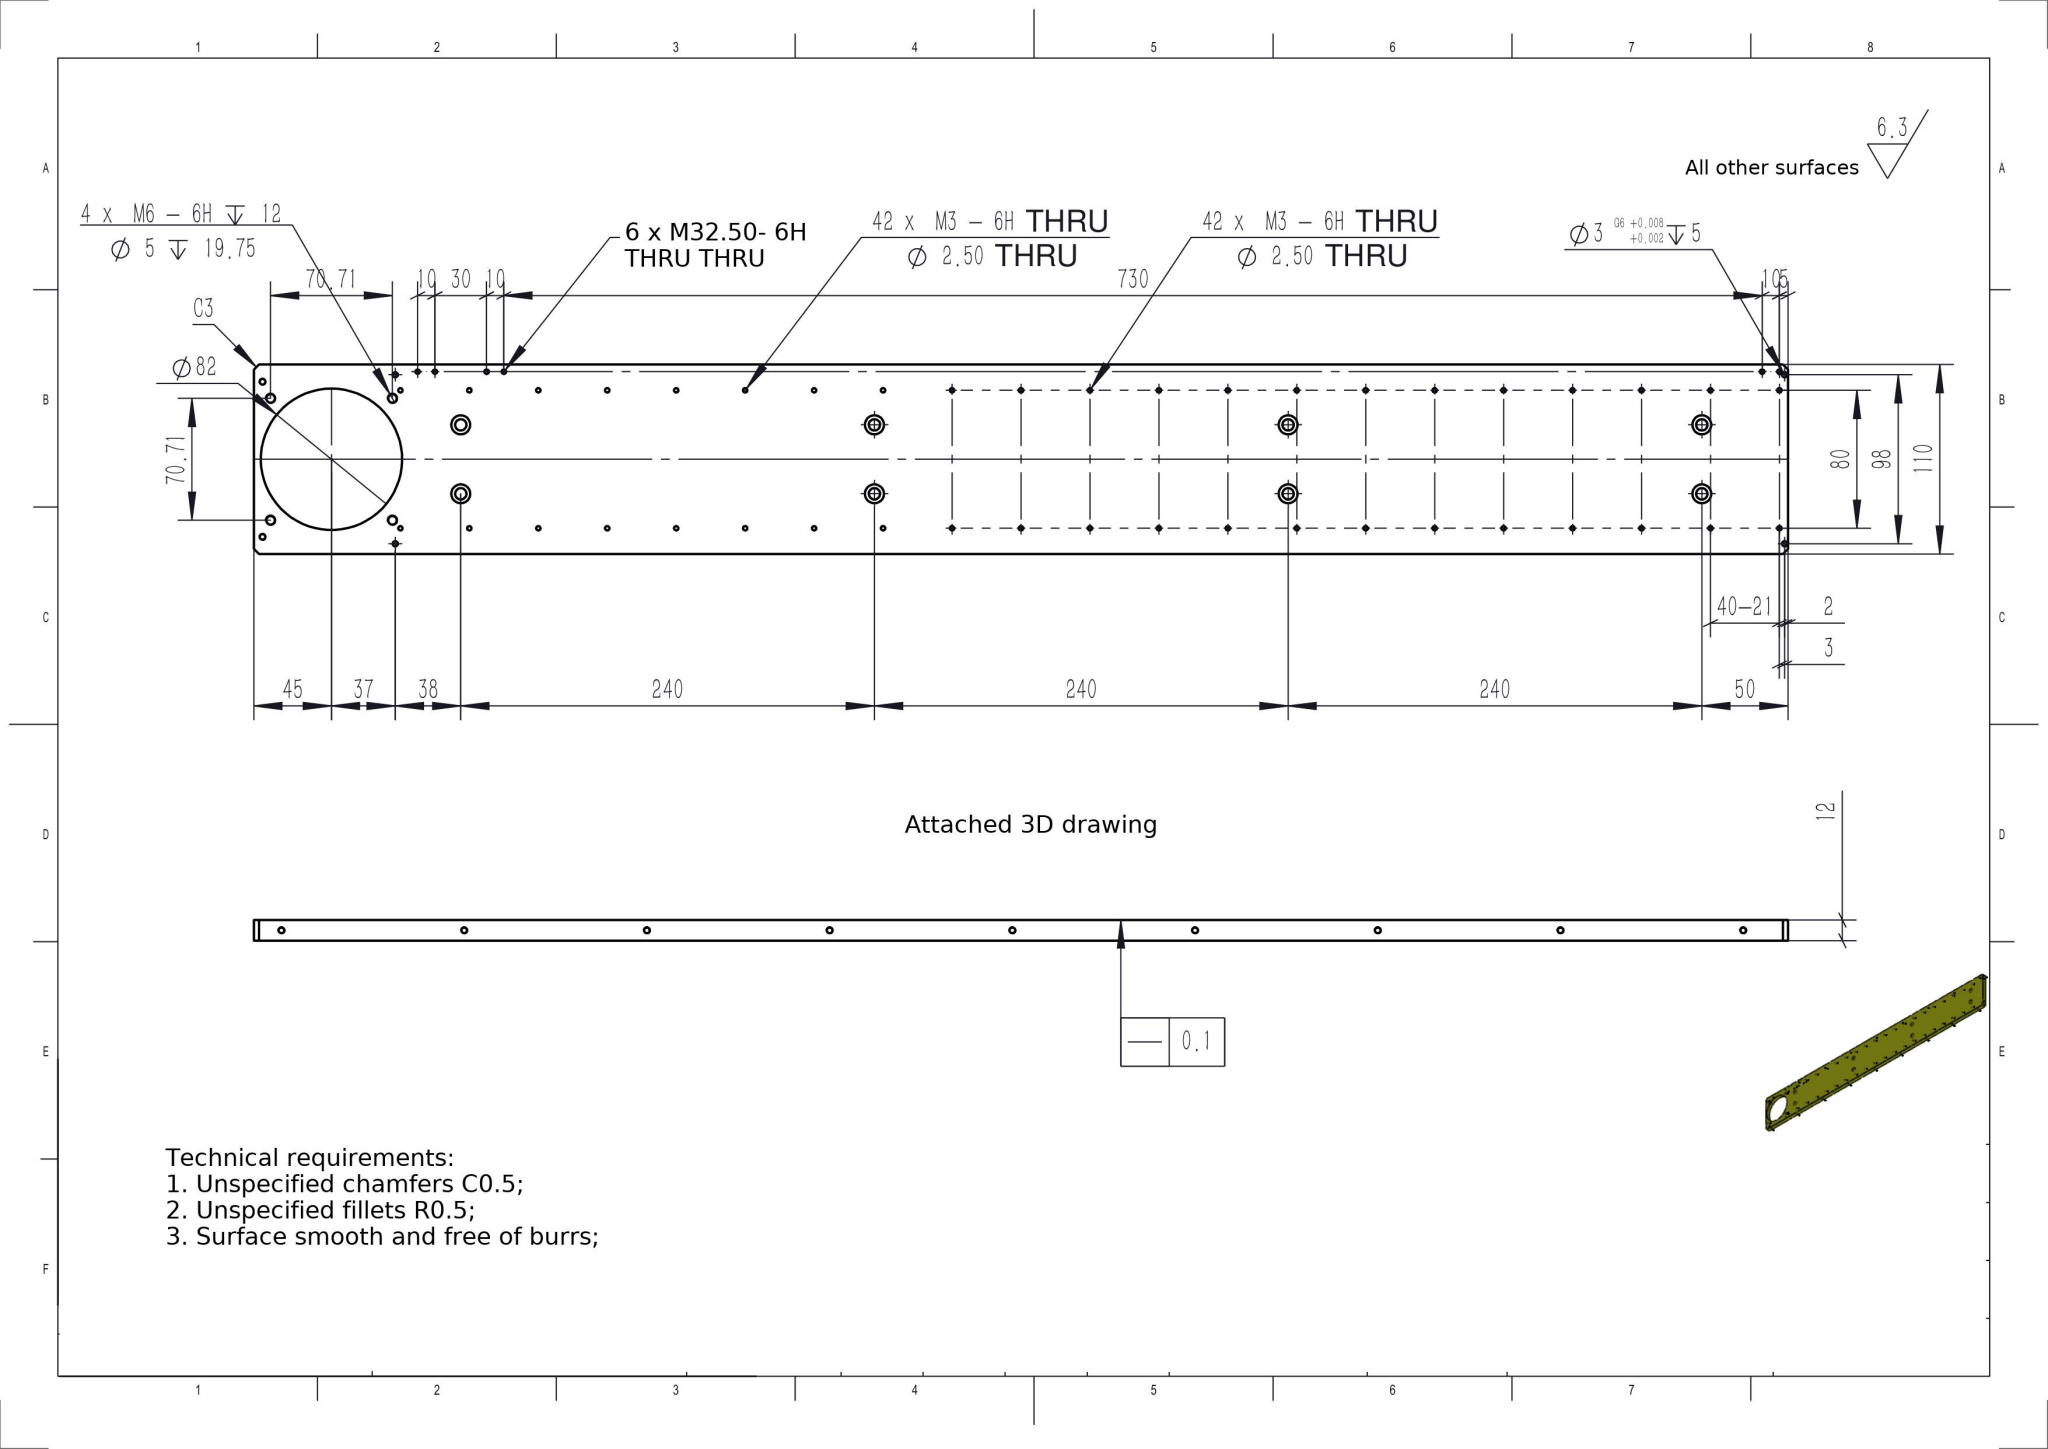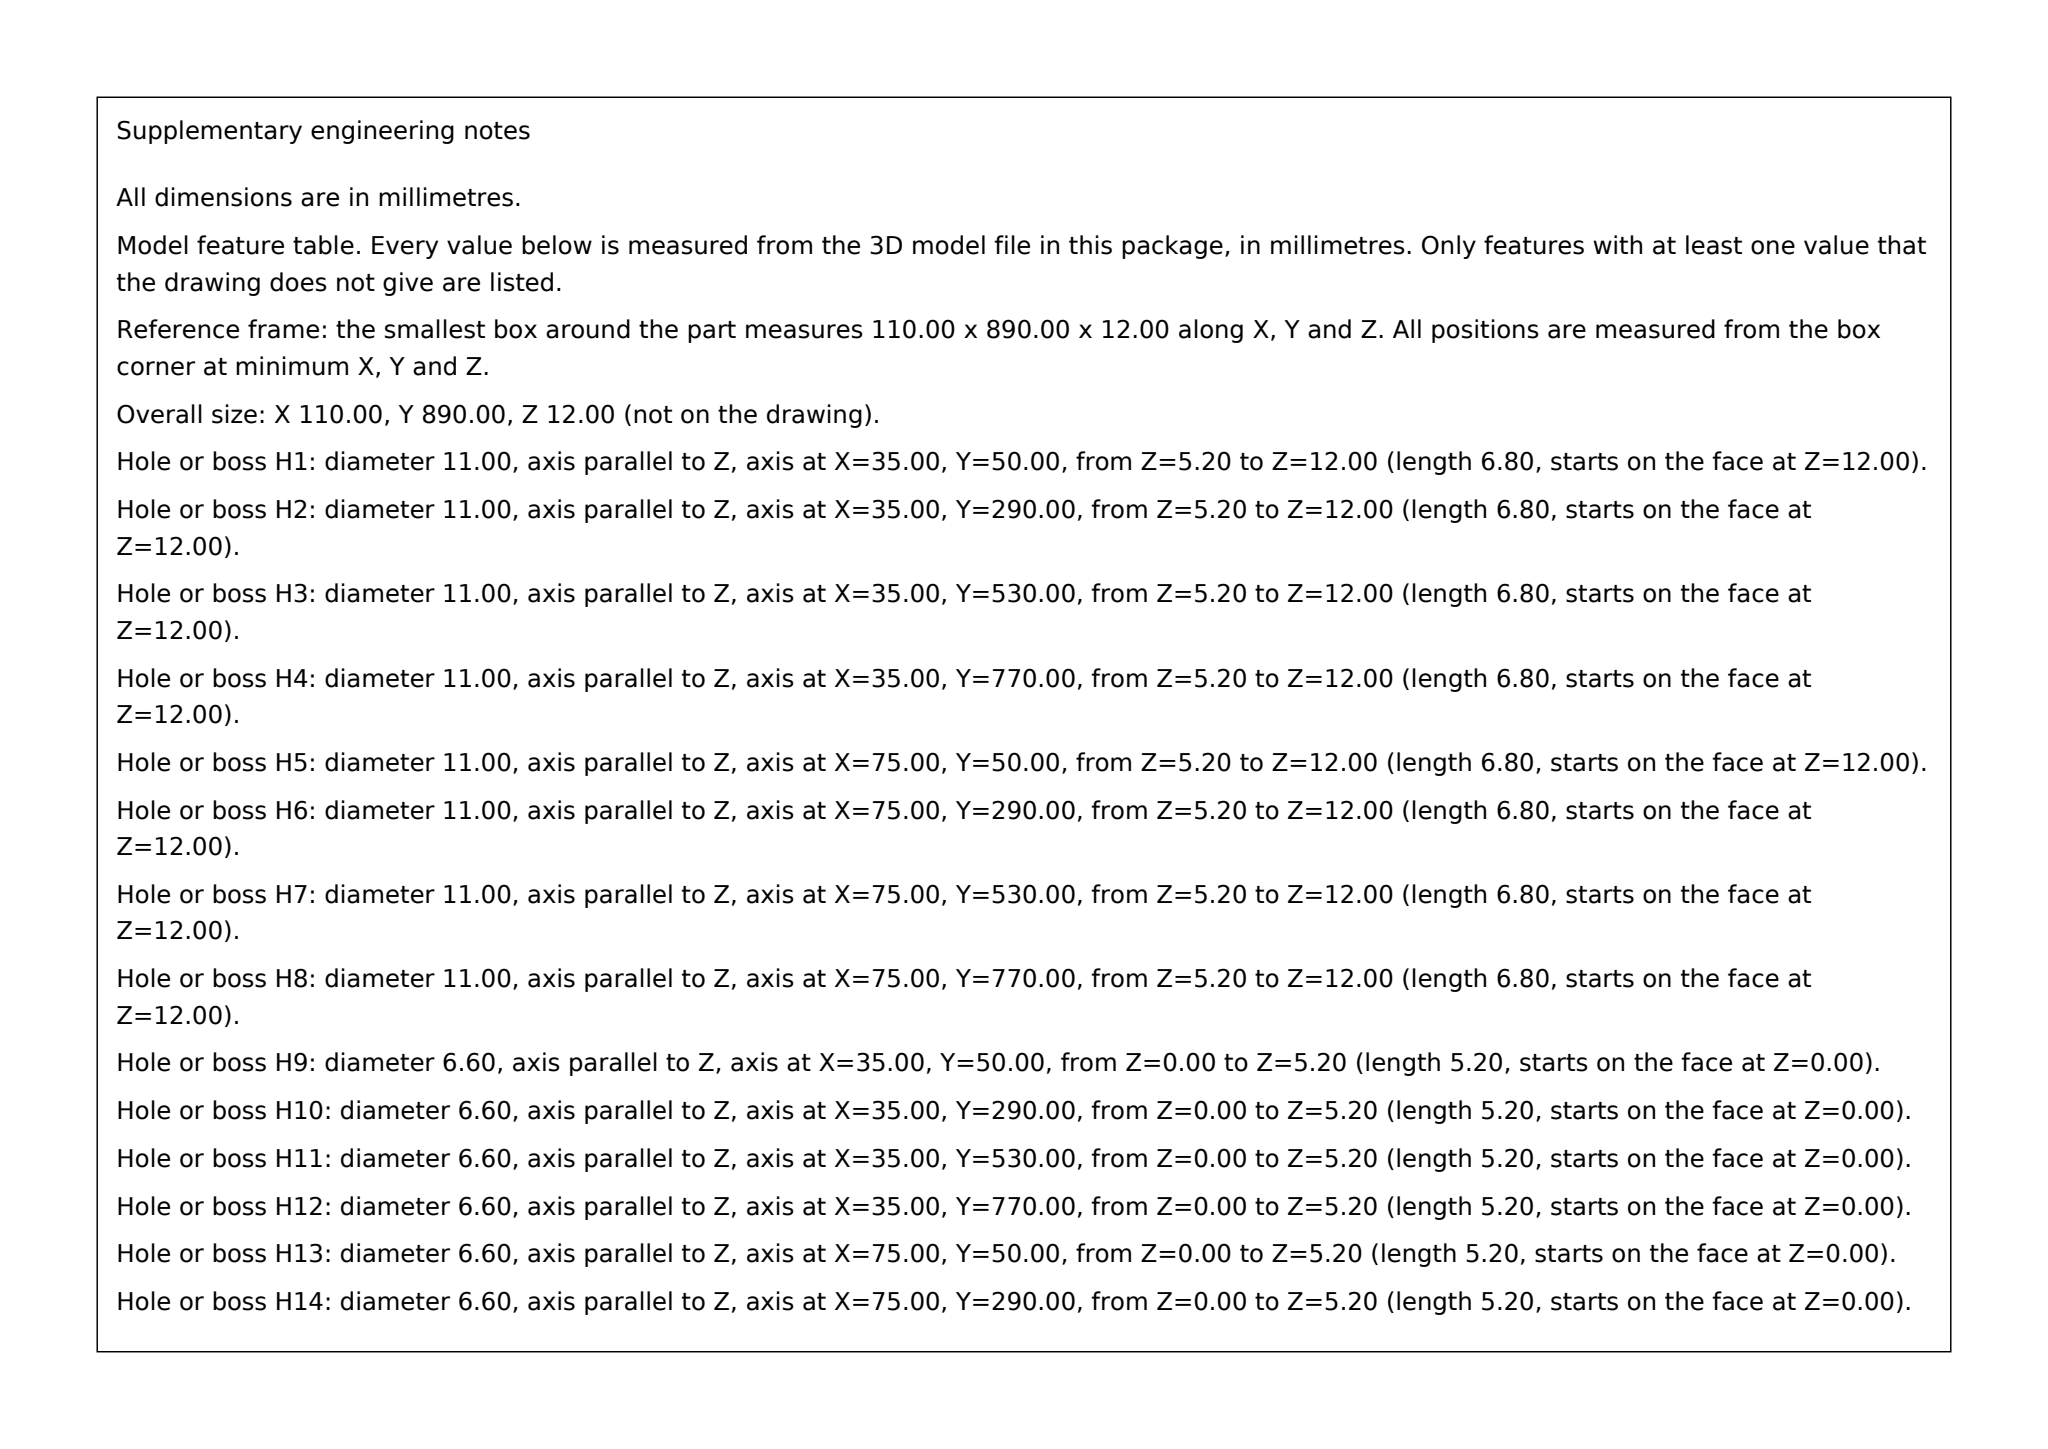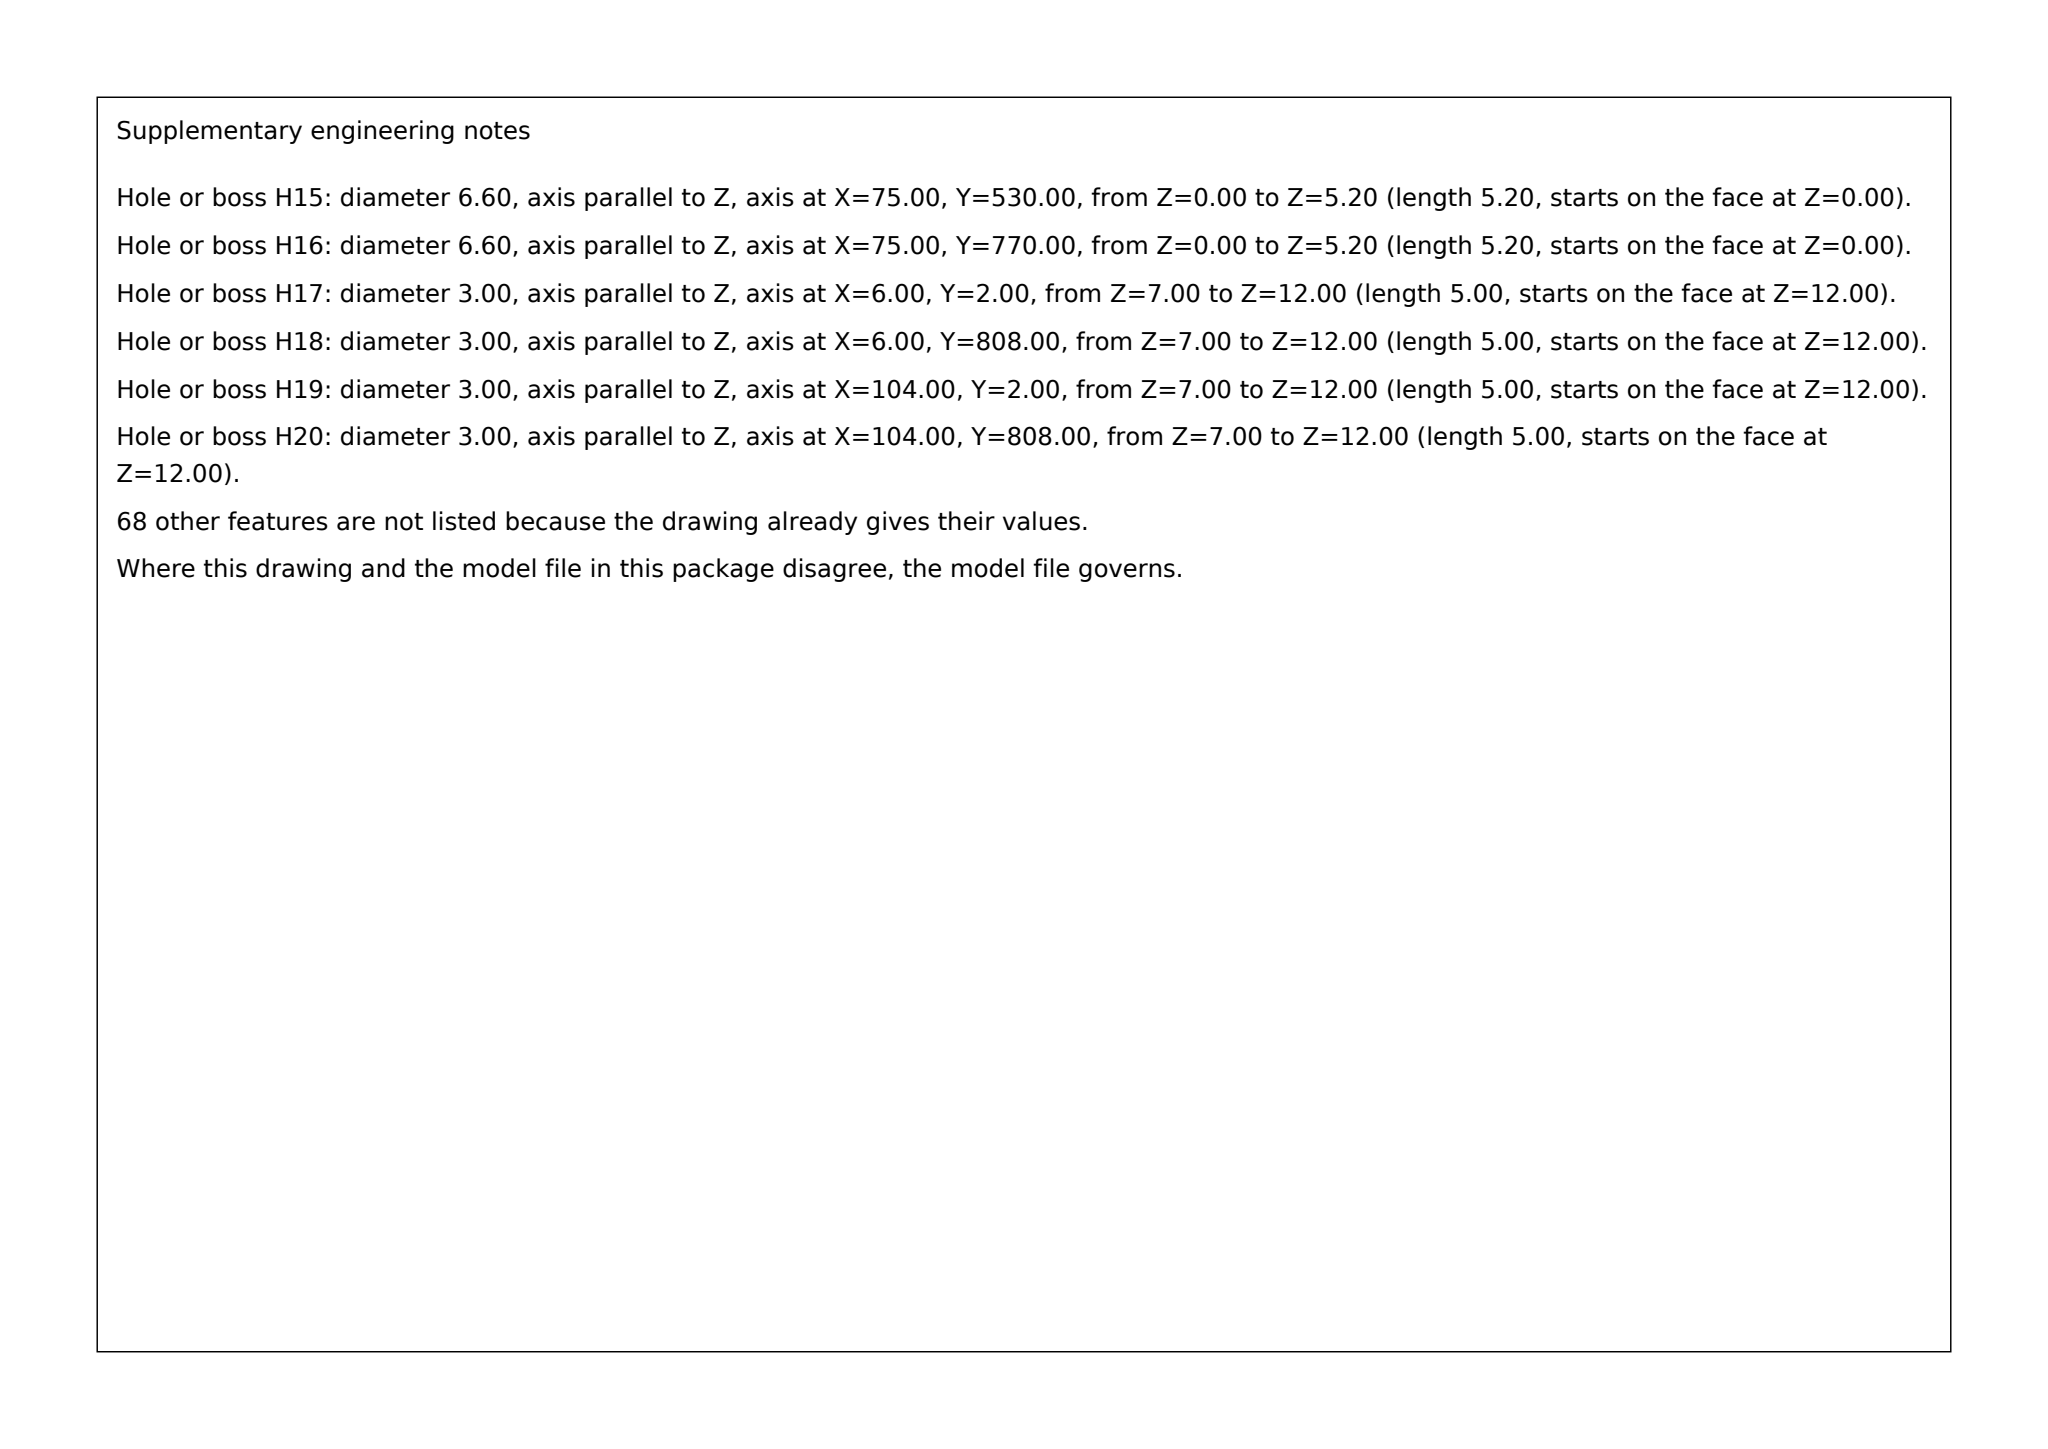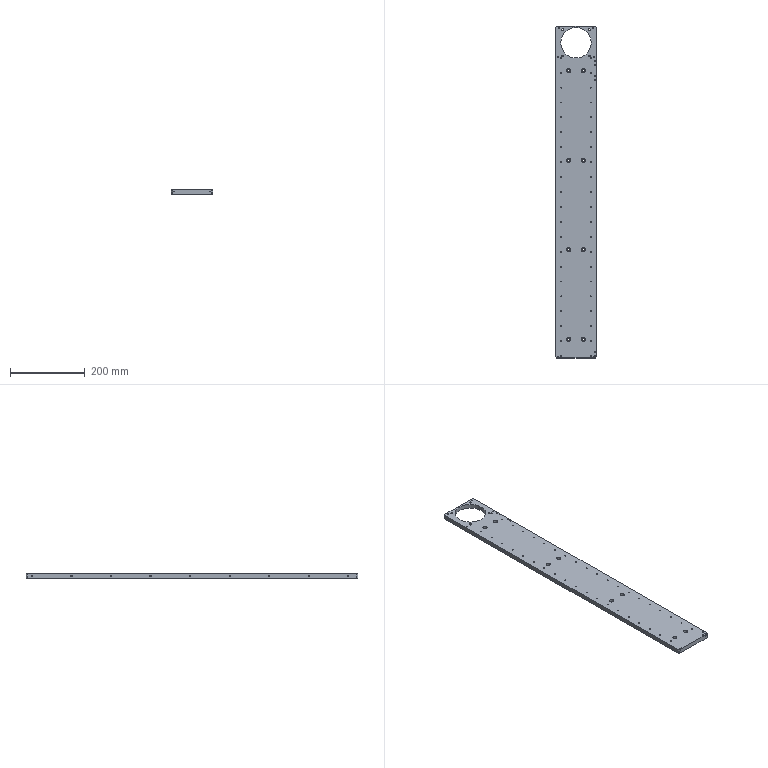Part | SolidWorks | mm | 1 solid | 244 faces | box 110 x 890 x 12 mm | volume 1099358 mm3 | cylinder 186 | cone 36 | plane 22 | commonest cylinder face diameters 2.5 x96 3.3 x40 11 x16 6.6 x16 5 x8 3 x8 82 x2
build123d program:
from build123d import *

# Parameters (mm, degrees)
SKETCH1_W                                         = 110
SKETCH1_H                                         = 890
BOSS_EXTRUDE1_DEPTH                               = 12
HOLE_SIZE_ACCORDING_TO_TYPE_OF_HEXAGO_D           = 6.6
HOLE_SIZE_ACCORDING_TO_TYPE_OF_HEXAGO_DEPTH       = 19.75
HOLE_SIZE_ACCORDING_TO_TYPE_OF_HEXAGO_CBORE_D     = 11
HOLE_SIZE_ACCORDING_TO_TYPE_OF_HEXAGO_CBORE_DEPTH = 6.8
HOLE_SIZE_ACCORDING_TO_TYPE_OF_HEXAGO_TIP         = 1.983
SKETCH7_R                                         = 1.5
CUT_EXTRUDE1_DEPTH                                = 5
M3_TAPPED_HOLE1_D                                 = 2.5
SKETCH12_R                                        = 41
CUT_EXTRUDE2_DEPTH                                = 449.547
M3_TAPPED_HOLE2_D                                 = 2.5
M6_TAPPED_HOLE1_D                                 = 5
M6_TAPPED_HOLE1_DEPTH                             = 19.75
M6_TAPPED_HOLE1_TIP                               = 1.502
CHAMFER1_SIZE                                     = 3
M4_TAPPED_HOLE1_D                                 = 3.3
LPATTERN1_COUNT                                   = 9
LPATTERN1_PITCH                                   = 106


with BuildPart() as part:
    # Sketch1 → Boss-Extrude1 (new body)
    with BuildSketch(Plane.XY):
        Rectangle(SKETCH1_W, SKETCH1_H)
    extrude(amount=BOSS_EXTRUDE1_DEPTH)

    # Hole Size _ according to_ Type of Hexago
    with Locations(Plane.XY.offset(12)):
        with Locations((-20, 85), (-20, -155), (20, -155), (20, 85), (20, -395), (-20, -395), (-20, 325), (20, 325)):
            CounterBoreHole(HOLE_SIZE_ACCORDING_TO_TYPE_OF_HEXAGO_D / 2, HOLE_SIZE_ACCORDING_TO_TYPE_OF_HEXAGO_CBORE_D / 2, HOLE_SIZE_ACCORDING_TO_TYPE_OF_HEXAGO_CBORE_DEPTH, depth=HOLE_SIZE_ACCORDING_TO_TYPE_OF_HEXAGO_DEPTH)
            with Locations((0, 0, -(HOLE_SIZE_ACCORDING_TO_TYPE_OF_HEXAGO_DEPTH + HOLE_SIZE_ACCORDING_TO_TYPE_OF_HEXAGO_TIP / 2))):  # 118° drill point
                Cone(0, HOLE_SIZE_ACCORDING_TO_TYPE_OF_HEXAGO_D / 2, HOLE_SIZE_ACCORDING_TO_TYPE_OF_HEXAGO_TIP, mode=Mode.SUBTRACT)

    # Sketch7 → Cut-Extrude1 (cut)
    with BuildSketch(Plane.XY.offset(12)):
        with Locations((-49, -443)):
            Circle(SKETCH7_R)
        with Locations((-49, 363)):
            Circle(SKETCH7_R)
        with Locations(Location((49, 363, 0), (0, 0, 180))):
            Circle(SKETCH7_R)
        with Locations(Location((49, -443, 0), (0, 0, 180))):
            Circle(SKETCH7_R)
    extrude(amount=-CUT_EXTRUDE1_DEPTH, mode=Mode.SUBTRACT)

    # M3 Tapped Hole1 (through all)
    with Locations(Plane.XY.offset(12)):
        with Locations((-40, -440), (40, -440), (-40, -400), (40, -400), (-40, -360), (40, -360), (-40, -320), (40, -320), (-40, -280), (40, -280), (-40, -240), (40, -240), (-40, -200), (40, -200), (-40, -160), (40, -160), (-40, -120), (40, -120), (-40, -80), (40, -80), (-40, -40), (40, -40), (-40, 0), (40, 0), (-40, 40), (40, 40), (-40, 80), (40, 80), (-40, 120), (40, 120), (-40, 160), (40, 160), (-40, 200), (40, 200), (-40, 240), (40, 240), (-40, 280), (40, 280), (-40, 320), (40, 320), (-40, 360), (40, 360)):
            Hole(M3_TAPPED_HOLE1_D / 2)

    # Sketch12 → Cut-Extrude2 (cut, through all)
    with BuildSketch(Plane.XY.offset(12)):
        with Locations((0, 400)):
            Circle(SKETCH12_R)
    extrude(amount=-CUT_EXTRUDE2_DEPTH, mode=Mode.SUBTRACT)

    # M3 Tapped Hole2 (through all)
    with Locations(Plane(origin=(0, 0, 0), x_dir=(-1, 0, 0), z_dir=(0, 0, -1))):
        with Locations((-50.8, -440), (-50.8, -430), (-50.8, 340), (-50.8, 350), (-50.8, 300), (-50.8, 310)):
            Hole(M3_TAPPED_HOLE2_D / 2)

    # M6 Tapped Hole1
    with Locations(Plane.XY.offset(12)):
        with Locations((-35.355, 435.355), (35.355, 435.355), (35.355, 364.645), (-35.355, 364.645)):
            Hole(M6_TAPPED_HOLE1_D / 2, depth=M6_TAPPED_HOLE1_DEPTH)
            with Locations((0, 0, -(M6_TAPPED_HOLE1_DEPTH + M6_TAPPED_HOLE1_TIP / 2))):  # 118° drill point
                Cone(0, M6_TAPPED_HOLE1_D / 2, M6_TAPPED_HOLE1_TIP, mode=Mode.SUBTRACT)

    # Chamfer1
    chamfer1_edges = [part.edges().sort_by_distance(p)[0] for p in [
        (55, -445, 6),
        (-55, -445, 6),
        (-55, 445, 6),
        (55, 445, 6),
    ]]
    chamfer(chamfer1_edges, length=CHAMFER1_SIZE)

    # M4 Tapped Hole1 (through all)
    with Locations(Plane.XY.offset(12)):
        with Locations((45, 440), (-45, 440)):
            Hole(M4_TAPPED_HOLE1_D / 2)

    # Sketch21 → M4 Tapped Hole2 (revolve, cut)
    with BuildSketch(Plane(origin=(55, 429, 6), x_dir=(0, 0, -1), z_dir=(0, 1, 0))):
        Polygon((0, 0), (0, 11.091), (1.65, 10.1), (1.65, 0), align=None)
    m4_tapped_hole2 = revolve(axis=Axis((61.35, 429, 6), (-1, 0, 0)), mode=Mode.SUBTRACT)

    # LPattern1: M4 Tapped Hole2 ×9
    with Locations(*[(0, -i * LPATTERN1_PITCH, 0) for i in range(1, LPATTERN1_COUNT)]):
        add(m4_tapped_hole2, mode=Mode.SUBTRACT)

    # Mirror1: M4 Tapped Hole2 across plane
    add(m4_tapped_hole2.mirror(Plane(origin=(-3, 0, 0), x_dir=(0, 0, 1), z_dir=(1, 0, 0))), mode=Mode.SUBTRACT)

    # Mirror1 copy 1 sketch → Mirror1 copy 1 (revolve, cut)
    with BuildSketch(Plane(origin=(-61, 323, 6), x_dir=(0, 0, -1), z_dir=(0, 1, 0))):
        Polygon((0, 0), (0, -11.091), (1.65, -10.1), (1.65, 0), align=None)
    revolve(axis=Axis((-67.35, 323, 6), (-1, 0, 0)), mode=Mode.SUBTRACT)

    # Mirror1 copy 2 sketch → Mirror1 copy 2 (revolve, cut)
    with BuildSketch(Plane(origin=(-61, 217, 6), x_dir=(0, 0, -1), z_dir=(0, 1, 0))):
        Polygon((0, 0), (0, -11.091), (1.65, -10.1), (1.65, 0), align=None)
    revolve(axis=Axis((-67.35, 217, 6), (-1, 0, 0)), mode=Mode.SUBTRACT)

    # Mirror1 copy 3 sketch → Mirror1 copy 3 (revolve, cut)
    with BuildSketch(Plane(origin=(-61, 111, 6), x_dir=(0, 0, -1), z_dir=(0, 1, 0))):
        Polygon((0, 0), (0, -11.091), (1.65, -10.1), (1.65, 0), align=None)
    revolve(axis=Axis((-67.35, 111, 6), (-1, 0, 0)), mode=Mode.SUBTRACT)

    # Mirror1 copy 4 sketch → Mirror1 copy 4 (revolve, cut)
    with BuildSketch(Plane(origin=(-61, 5, 6), x_dir=(0, 0, -1), z_dir=(0, 1, 0))):
        Polygon((0, 0), (0, -11.091), (1.65, -10.1), (1.65, 0), align=None)
    revolve(axis=Axis((-67.35, 5, 6), (-1, 0, 0)), mode=Mode.SUBTRACT)

    # Mirror1 copy 5 sketch → Mirror1 copy 5 (revolve, cut)
    with BuildSketch(Plane(origin=(-61, -101, 6), x_dir=(0, 0, -1), z_dir=(0, 1, 0))):
        Polygon((0, 0), (0, -11.091), (1.65, -10.1), (1.65, 0), align=None)
    revolve(axis=Axis((-67.35, -101, 6), (-1, 0, 0)), mode=Mode.SUBTRACT)

    # Mirror1 copy 6 sketch → Mirror1 copy 6 (revolve, cut)
    with BuildSketch(Plane(origin=(-61, -207, 6), x_dir=(0, 0, -1), z_dir=(0, 1, 0))):
        Polygon((0, 0), (0, -11.091), (1.65, -10.1), (1.65, 0), align=None)
    revolve(axis=Axis((-67.35, -207, 6), (-1, 0, 0)), mode=Mode.SUBTRACT)

    # Mirror1 copy 7 sketch → Mirror1 copy 7 (revolve, cut)
    with BuildSketch(Plane(origin=(-61, -313, 6), x_dir=(0, 0, -1), z_dir=(0, 1, 0))):
        Polygon((0, 0), (0, -11.091), (1.65, -10.1), (1.65, 0), align=None)
    revolve(axis=Axis((-67.35, -313, 6), (-1, 0, 0)), mode=Mode.SUBTRACT)

    # Mirror1 copy 8 sketch → Mirror1 copy 8 (revolve, cut)
    with BuildSketch(Plane(origin=(-61, -419, 6), x_dir=(0, 0, -1), z_dir=(0, 1, 0))):
        Polygon((0, 0), (0, -11.091), (1.65, -10.1), (1.65, 0), align=None)
    revolve(axis=Axis((-67.35, -419, 6), (-1, 0, 0)), mode=Mode.SUBTRACT)


solid = part.part